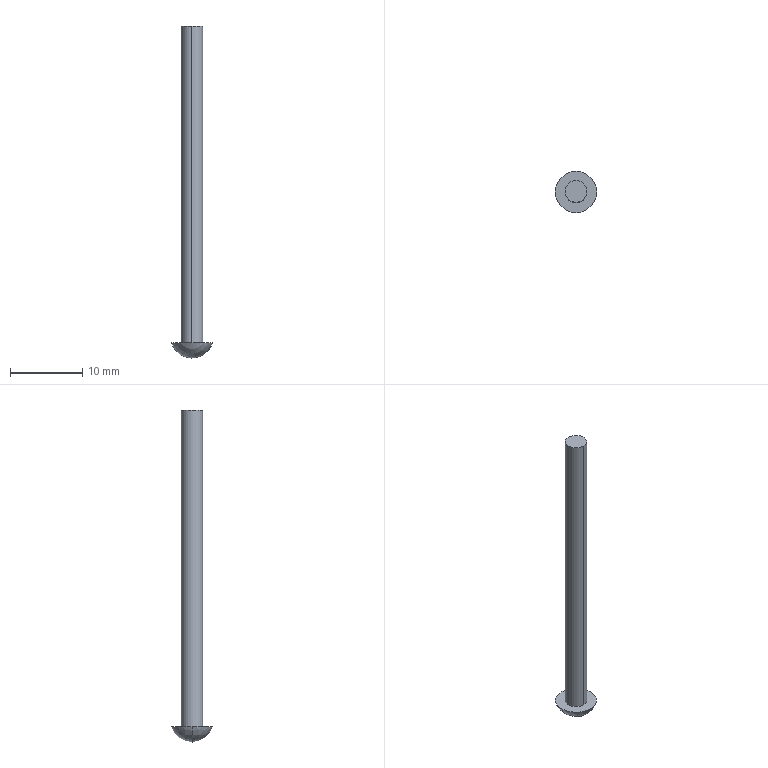Component | SolidWorks | 21FuelTankCapPin-1 | 1 solid | 6 faces | box 5.72 x 5.72 x 46.1 mm | volume 343 mm3 | cylinder 2 | sphere 2 | plane 2 | commonest cylinder face diameters 3 x2
build123d program:
from build123d import *

# Parameters (mm, degrees)
SKETCH43_R          = 1.5
BOSS_EXTRUDE9_DEPTH = 44


with BuildPart() as part:
    # Sketch41 → Revolve3 (revolve)
    with BuildSketch(Plane.XY, mode=Mode.PRIVATE) as revolve3_sk:
        with BuildLine():
            Line((0, 2.1), (0, 0))
            Line((0, 0), (-2.862, 0))
            ThreePointArc((-2.862, 0), (-1.775, 1.519), (0, 2.1))
        make_face()
    revolve(revolve3_sk.sketch.rotate(Axis((0, 2.1, 0), (0, -1, 0)), 180), axis=Axis((0, 2.1, 0), (0, -1, 0)))

    # Sketch43 → Boss-Extrude9 (add)
    with BuildSketch(Plane.XZ):
        with Locations(Location((0, 0, 0), (0, 0, 270))):
            Circle(SKETCH43_R)
    extrude(amount=BOSS_EXTRUDE9_DEPTH)


solid = part.part

# Placed as in the assembly
solid = solid.moved(Location((82.885, 376.809, 492), (-90, 0, 0)))
STEP:
#1=COLOUR_RGB('',0.7922,0.8196,0.9333);
#2=FILL_AREA_STYLE_COLOUR('',#1);
#3=FILL_AREA_STYLE('',(#2));
#4=SURFACE_STYLE_FILL_AREA(#3);
#5=SURFACE_SIDE_STYLE('',(#4));
#6=SURFACE_STYLE_USAGE(.BOTH.,#5);
#7=PRESENTATION_STYLE_ASSIGNMENT((#6));
#8=CARTESIAN_POINT('',(3.263,14.776,21.102));
#9=VERTEX_POINT('',#8);
#10=CARTESIAN_POINT('',(3.263,14.894,21.102));
#11=VERTEX_POINT('',#10);
#12=CARTESIAN_POINT('',(3.263,14.835,21.102));
#13=DIRECTION('',(0.,0.,1.));
#14=DIRECTION('',(0.,-1.,0.));
#15=AXIS2_PLACEMENT_3D('',#12,#13,#14);
#16=CIRCLE('',#15,0.05906);
#17=EDGE_CURVE('',#9,#11,#16,.T.);
#18=ORIENTED_EDGE('',*,*,#17,.F.);
#19=CARTESIAN_POINT('',(3.263,14.776,19.37));
#20=VERTEX_POINT('',#19);
#21=CARTESIAN_POINT('',(3.263,14.776,21.102));
#22=DIRECTION('',(0.,0.,-1.));
#23=VECTOR('',#22,39.37);
#24=LINE('',#21,#23);
#25=EDGE_CURVE('',#9,#20,#24,.T.);
#26=ORIENTED_EDGE('',*,*,#25,.T.);
#27=CARTESIAN_POINT('',(3.263,14.894,19.37));
#28=VERTEX_POINT('',#27);
#29=CARTESIAN_POINT('',(3.263,14.835,19.37));
#30=DIRECTION('',(0.,0.,1.));
#31=DIRECTION('',(0.,-1.,0.));
#32=AXIS2_PLACEMENT_3D('',#29,#30,#31);
#33=CIRCLE('',#32,0.05906);
#34=EDGE_CURVE('',#20,#28,#33,.T.);
#35=ORIENTED_EDGE('',*,*,#34,.T.);
#36=CARTESIAN_POINT('',(3.263,14.894,21.102));
#37=DIRECTION('',(0.,0.,-1.));
#38=VECTOR('',#37,39.37);
#39=LINE('',#36,#38);
#40=EDGE_CURVE('',#11,#28,#39,.T.);
#41=ORIENTED_EDGE('',*,*,#40,.F.);
#42=EDGE_LOOP('',(#18,#26,#35,#41));
#43=FACE_OUTER_BOUND('',#42,.T.);
#44=CARTESIAN_POINT('',(3.263,14.835,21.102));
#45=DIRECTION('',(0.,0.,-1.));
#46=DIRECTION('',(0.,1.,0.));
#47=AXIS2_PLACEMENT_3D('',#44,#45,#46);
#48=CYLINDRICAL_SURFACE('',#47,0.05906);
#49=ADVANCED_FACE('',(#43),#48,.T.);
#50=CARTESIAN_POINT('',(3.376,14.835,19.37));
#51=VERTEX_POINT('',#50);
#52=CARTESIAN_POINT('',(3.151,14.835,19.37));
#53=VERTEX_POINT('',#52);
#54=CARTESIAN_POINT('',(3.263,14.835,19.37));
#55=DIRECTION('',(0.,0.,-1.));
#56=DIRECTION('',(0.,1.,0.));
#57=AXIS2_PLACEMENT_3D('',#54,#55,#56);
#58=CIRCLE('',#57,0.1127);
#59=EDGE_CURVE('',#51,#53,#58,.T.);
#60=ORIENTED_EDGE('',*,*,#59,.T.);
#61=CARTESIAN_POINT('',(3.263,14.835,19.287));
#62=VERTEX_POINT('',#61);
#63=CARTESIAN_POINT('',(3.263,14.835,19.406));
#64=DIRECTION('',(0.,-1.,0.));
#65=DIRECTION('',(1.,0.,0.));
#66=AXIS2_PLACEMENT_3D('',#63,#64,#65);
#67=CIRCLE('',#66,0.1181);
#68=EDGE_CURVE('',#53,#62,#67,.T.);
#69=ORIENTED_EDGE('',*,*,#68,.T.);
#70=CARTESIAN_POINT('',(3.263,14.835,19.406));
#71=DIRECTION('',(0.,1.,0.));
#72=DIRECTION('',(0.,0.,1.));
#73=AXIS2_PLACEMENT_3D('',#70,#71,#72);
#74=CIRCLE('',#73,0.1181);
#75=EDGE_CURVE('',#51,#62,#74,.T.);
#76=ORIENTED_EDGE('',*,*,#75,.F.);
#77=EDGE_LOOP('',(#60,#69,#76));
#78=FACE_OUTER_BOUND('',#77,.T.);
#79=CARTESIAN_POINT('',(3.263,14.835,19.406));
#80=DIRECTION('',(0.,-1.,0.));
#81=DIRECTION('',(1.,0.,0.));
#82=AXIS2_PLACEMENT_3D('',#79,#80,#81);
#83=SPHERICAL_SURFACE('',#82,0.1181);
#84=ADVANCED_FACE('',(#78),#83,.T.);
#85=ORIENTED_EDGE('',*,*,#68,.F.);
#86=CARTESIAN_POINT('',(3.263,14.835,19.37));
#87=DIRECTION('',(0.,0.,-1.));
#88=DIRECTION('',(0.,1.,0.));
#89=AXIS2_PLACEMENT_3D('',#86,#87,#88);
#90=CIRCLE('',#89,0.1127);
#91=EDGE_CURVE('',#53,#51,#90,.T.);
#92=ORIENTED_EDGE('',*,*,#91,.T.);
#93=ORIENTED_EDGE('',*,*,#75,.T.);
#94=EDGE_LOOP('',(#85,#92,#93));
#95=FACE_OUTER_BOUND('',#94,.T.);
#96=CARTESIAN_POINT('',(3.263,14.835,19.406));
#97=DIRECTION('',(0.,-1.,0.));
#98=DIRECTION('',(1.,0.,0.));
#99=AXIS2_PLACEMENT_3D('',#96,#97,#98);
#100=SPHERICAL_SURFACE('',#99,0.1181);
#101=ADVANCED_FACE('',(#95),#100,.T.);
#102=CARTESIAN_POINT('',(3.263,14.835,19.37));
#103=DIRECTION('',(0.,0.,1.));
#104=DIRECTION('',(0.,-1.,0.));
#105=AXIS2_PLACEMENT_3D('',#102,#103,#104);
#106=CIRCLE('',#105,0.05906);
#107=EDGE_CURVE('',#28,#20,#106,.T.);
#108=ORIENTED_EDGE('',*,*,#107,.F.);
#109=ORIENTED_EDGE('',*,*,#34,.F.);
#110=EDGE_LOOP('',(#108,#109));
#111=FACE_BOUND('',#110,.T.);
#112=ORIENTED_EDGE('',*,*,#59,.F.);
#113=ORIENTED_EDGE('',*,*,#91,.F.);
#114=EDGE_LOOP('',(#112,#113));
#115=FACE_OUTER_BOUND('',#114,.T.);
#116=CARTESIAN_POINT('',(3.263,14.835,19.37));
#117=DIRECTION('',(0.,0.,1.));
#118=DIRECTION('',(0.,-1.,0.));
#119=AXIS2_PLACEMENT_3D('',#116,#117,#118);
#120=PLANE('',#119);
#121=ADVANCED_FACE('',(#111,#115),#120,.T.);
#122=ORIENTED_EDGE('',*,*,#25,.F.);
#123=CARTESIAN_POINT('',(3.263,14.835,21.102));
#124=DIRECTION('',(0.,0.,1.));
#125=DIRECTION('',(0.,-1.,0.));
#126=AXIS2_PLACEMENT_3D('',#123,#124,#125);
#127=CIRCLE('',#126,0.05906);
#128=EDGE_CURVE('',#11,#9,#127,.T.);
#129=ORIENTED_EDGE('',*,*,#128,.F.);
#130=ORIENTED_EDGE('',*,*,#40,.T.);
#131=ORIENTED_EDGE('',*,*,#107,.T.);
#132=EDGE_LOOP('',(#122,#129,#130,#131));
#133=FACE_OUTER_BOUND('',#132,.T.);
#134=CARTESIAN_POINT('',(3.263,14.835,21.102));
#135=DIRECTION('',(0.,0.,-1.));
#136=DIRECTION('',(0.,1.,0.));
#137=AXIS2_PLACEMENT_3D('',#134,#135,#136);
#138=CYLINDRICAL_SURFACE('',#137,0.05906);
#139=ADVANCED_FACE('',(#133),#138,.T.);
#140=ORIENTED_EDGE('',*,*,#128,.T.);
#141=ORIENTED_EDGE('',*,*,#17,.T.);
#142=EDGE_LOOP('',(#140,#141));
#143=FACE_OUTER_BOUND('',#142,.T.);
#144=CARTESIAN_POINT('',(3.263,14.835,21.102));
#145=DIRECTION('',(0.,0.,1.));
#146=DIRECTION('',(0.,-1.,0.));
#147=AXIS2_PLACEMENT_3D('',#144,#145,#146);
#148=PLANE('',#147);
#149=ADVANCED_FACE('',(#143),#148,.T.);
#150=CLOSED_SHELL('',(#49,#84,#101,#121,#139,#149));
#151=MANIFOLD_SOLID_BREP('',#150);
#152=STYLED_ITEM('',(#7),#151);
#153=PRESENTATION_LAYER_ASSIGNMENT('','',(#152));
#154=(LENGTH_UNIT()NAMED_UNIT(*)SI_UNIT($,.METRE.));
#155=LENGTH_MEASURE_WITH_UNIT(LENGTH_MEASURE(0.0254),#154);
#156=DIMENSIONAL_EXPONENTS(1.,0.,0.,0.,0.,0.,0.);
#157=(CONVERSION_BASED_UNIT('',#155)LENGTH_UNIT()NAMED_UNIT(#156));
#158=UNCERTAINTY_MEASURE_WITH_UNIT(LENGTH_MEASURE(0.00001),#157,'','');
#159=(NAMED_UNIT(*)PLANE_ANGLE_UNIT()SI_UNIT($,.RADIAN.));
#160=(NAMED_UNIT(*)SI_UNIT($,.STERADIAN.)SOLID_ANGLE_UNIT());
#161=(GEOMETRIC_REPRESENTATION_CONTEXT(3)GLOBAL_UNCERTAINTY_ASSIGNED_CONTEXT((#158))GLOBAL_UNIT_ASSIGNED_CONTEXT((#157,#159,#160))REPRESENTATION_CONTEXT('',''));
#162=MECHANICAL_DESIGN_GEOMETRIC_PRESENTATION_REPRESENTATION('',(#152),#161);
#163=CARTESIAN_POINT('',(0.,0.,0.));
#164=DIRECTION('',(0.,0.,1.));
#165=DIRECTION('',(1.,0.,0.));
#166=AXIS2_PLACEMENT_3D('',#163,#164,#165);
#167=(LENGTH_UNIT()NAMED_UNIT(*)SI_UNIT($,.METRE.));
#168=LENGTH_MEASURE_WITH_UNIT(LENGTH_MEASURE(0.0254),#167);
#169=DIMENSIONAL_EXPONENTS(1.,0.,0.,0.,0.,0.,0.);
#170=(CONVERSION_BASED_UNIT('',#168)LENGTH_UNIT()NAMED_UNIT(#169));
#171=UNCERTAINTY_MEASURE_WITH_UNIT(LENGTH_MEASURE(0.00001),#170,'','');
#172=(NAMED_UNIT(*)PLANE_ANGLE_UNIT()SI_UNIT($,.RADIAN.));
#173=(NAMED_UNIT(*)SI_UNIT($,.STERADIAN.)SOLID_ANGLE_UNIT());
#174=(GEOMETRIC_REPRESENTATION_CONTEXT(3)GLOBAL_UNCERTAINTY_ASSIGNED_CONTEXT((#171))GLOBAL_UNIT_ASSIGNED_CONTEXT((#170,#172,#173))REPRESENTATION_CONTEXT('',''));
#175=ADVANCED_BREP_SHAPE_REPRESENTATION('',(#151,#166),#174);